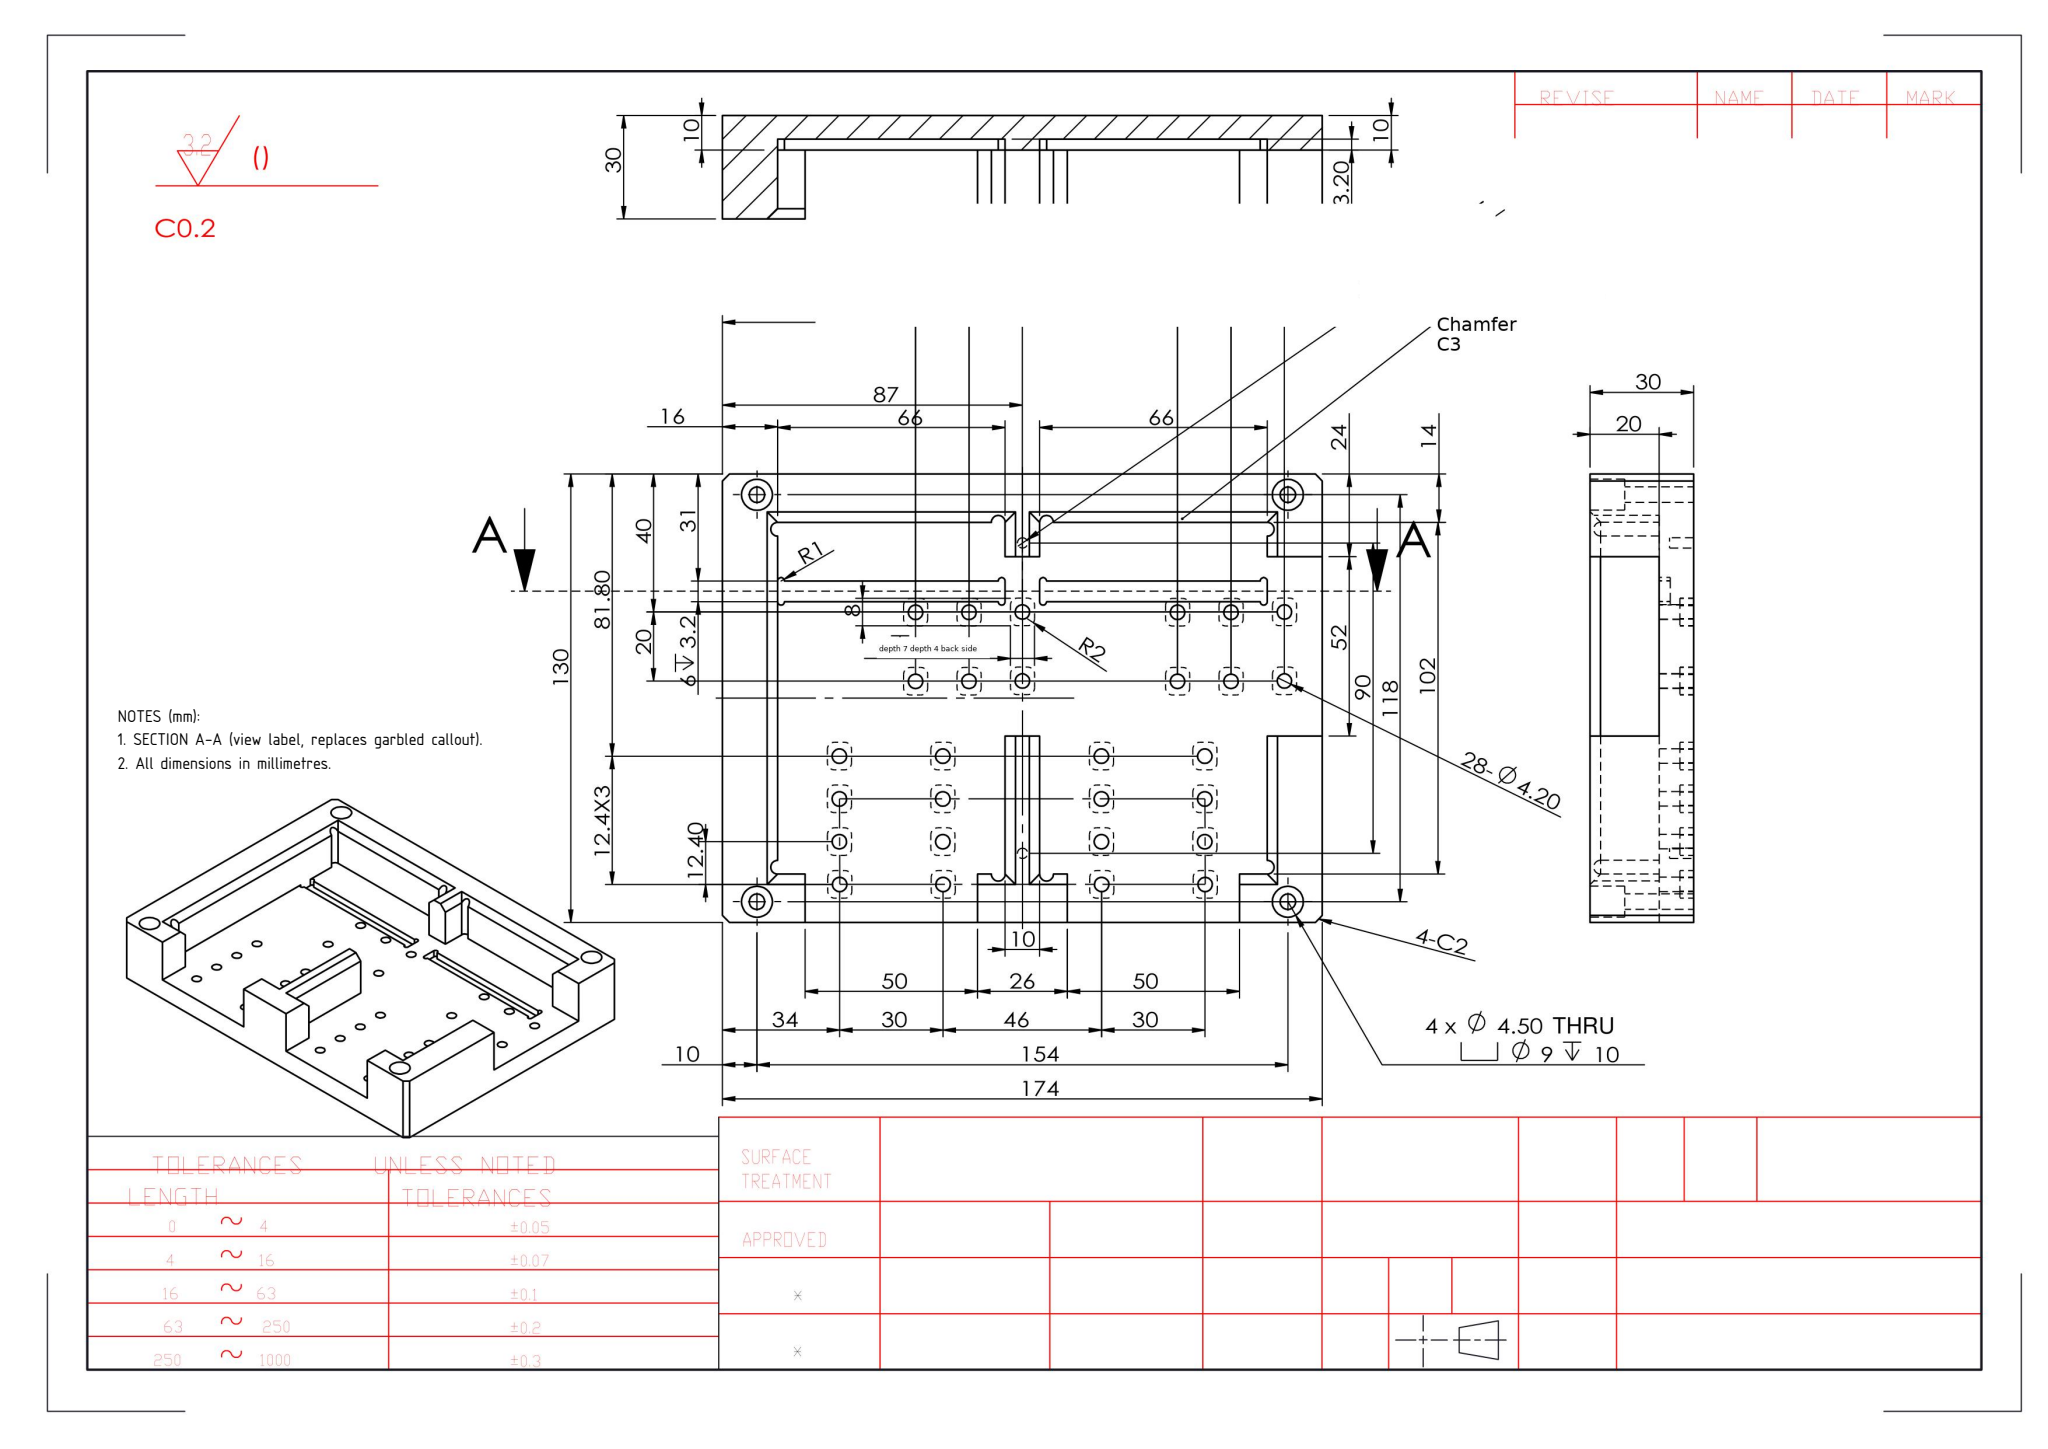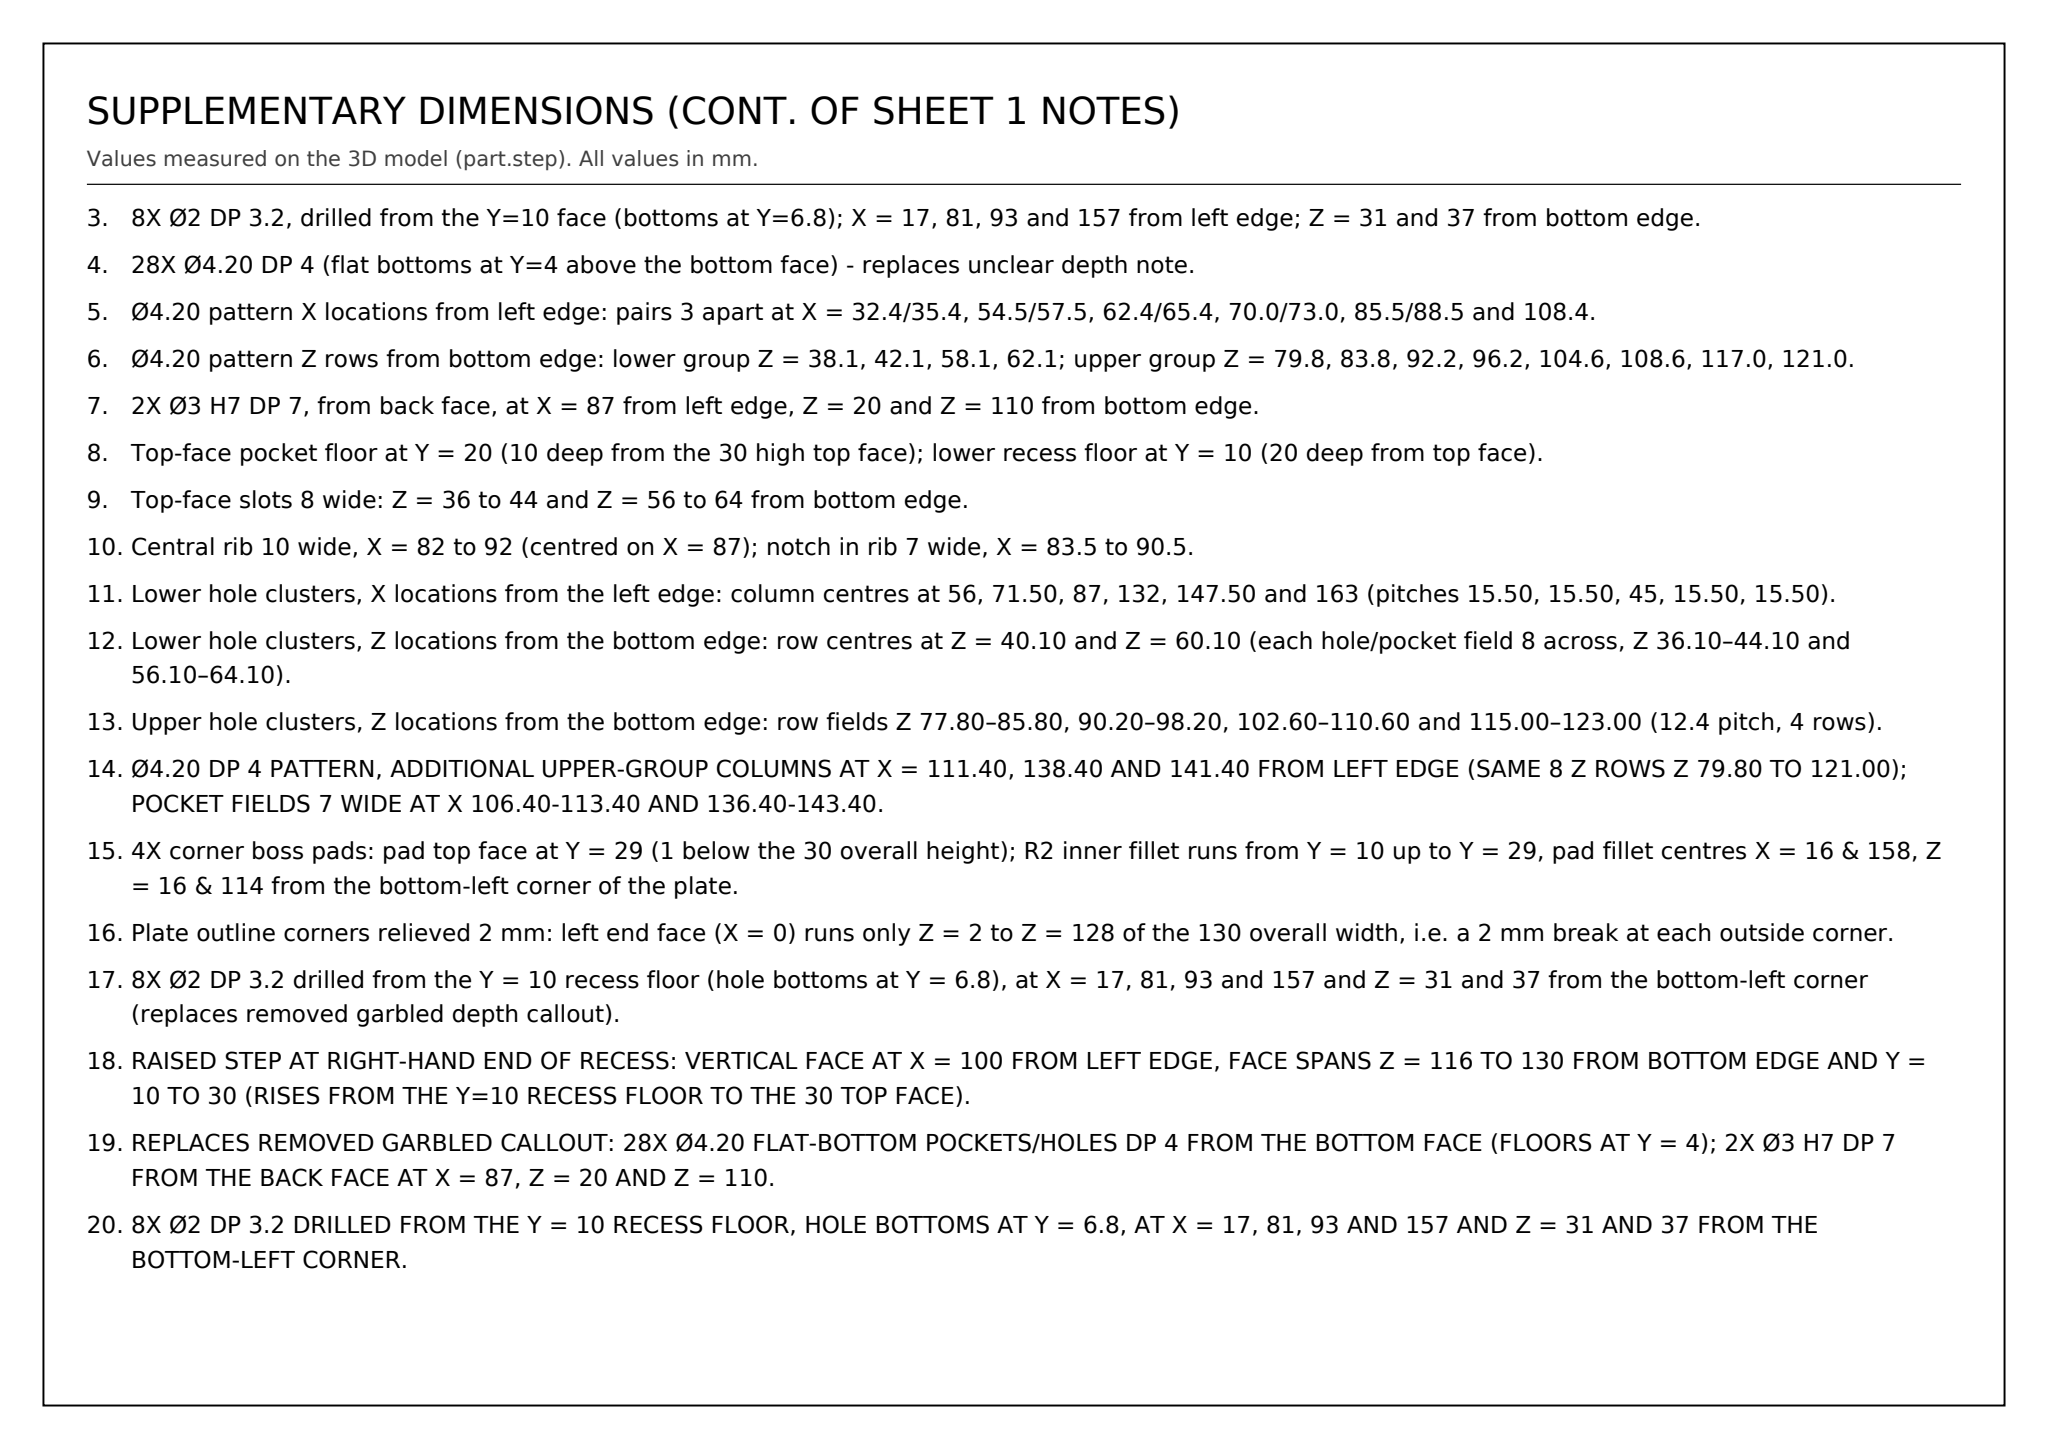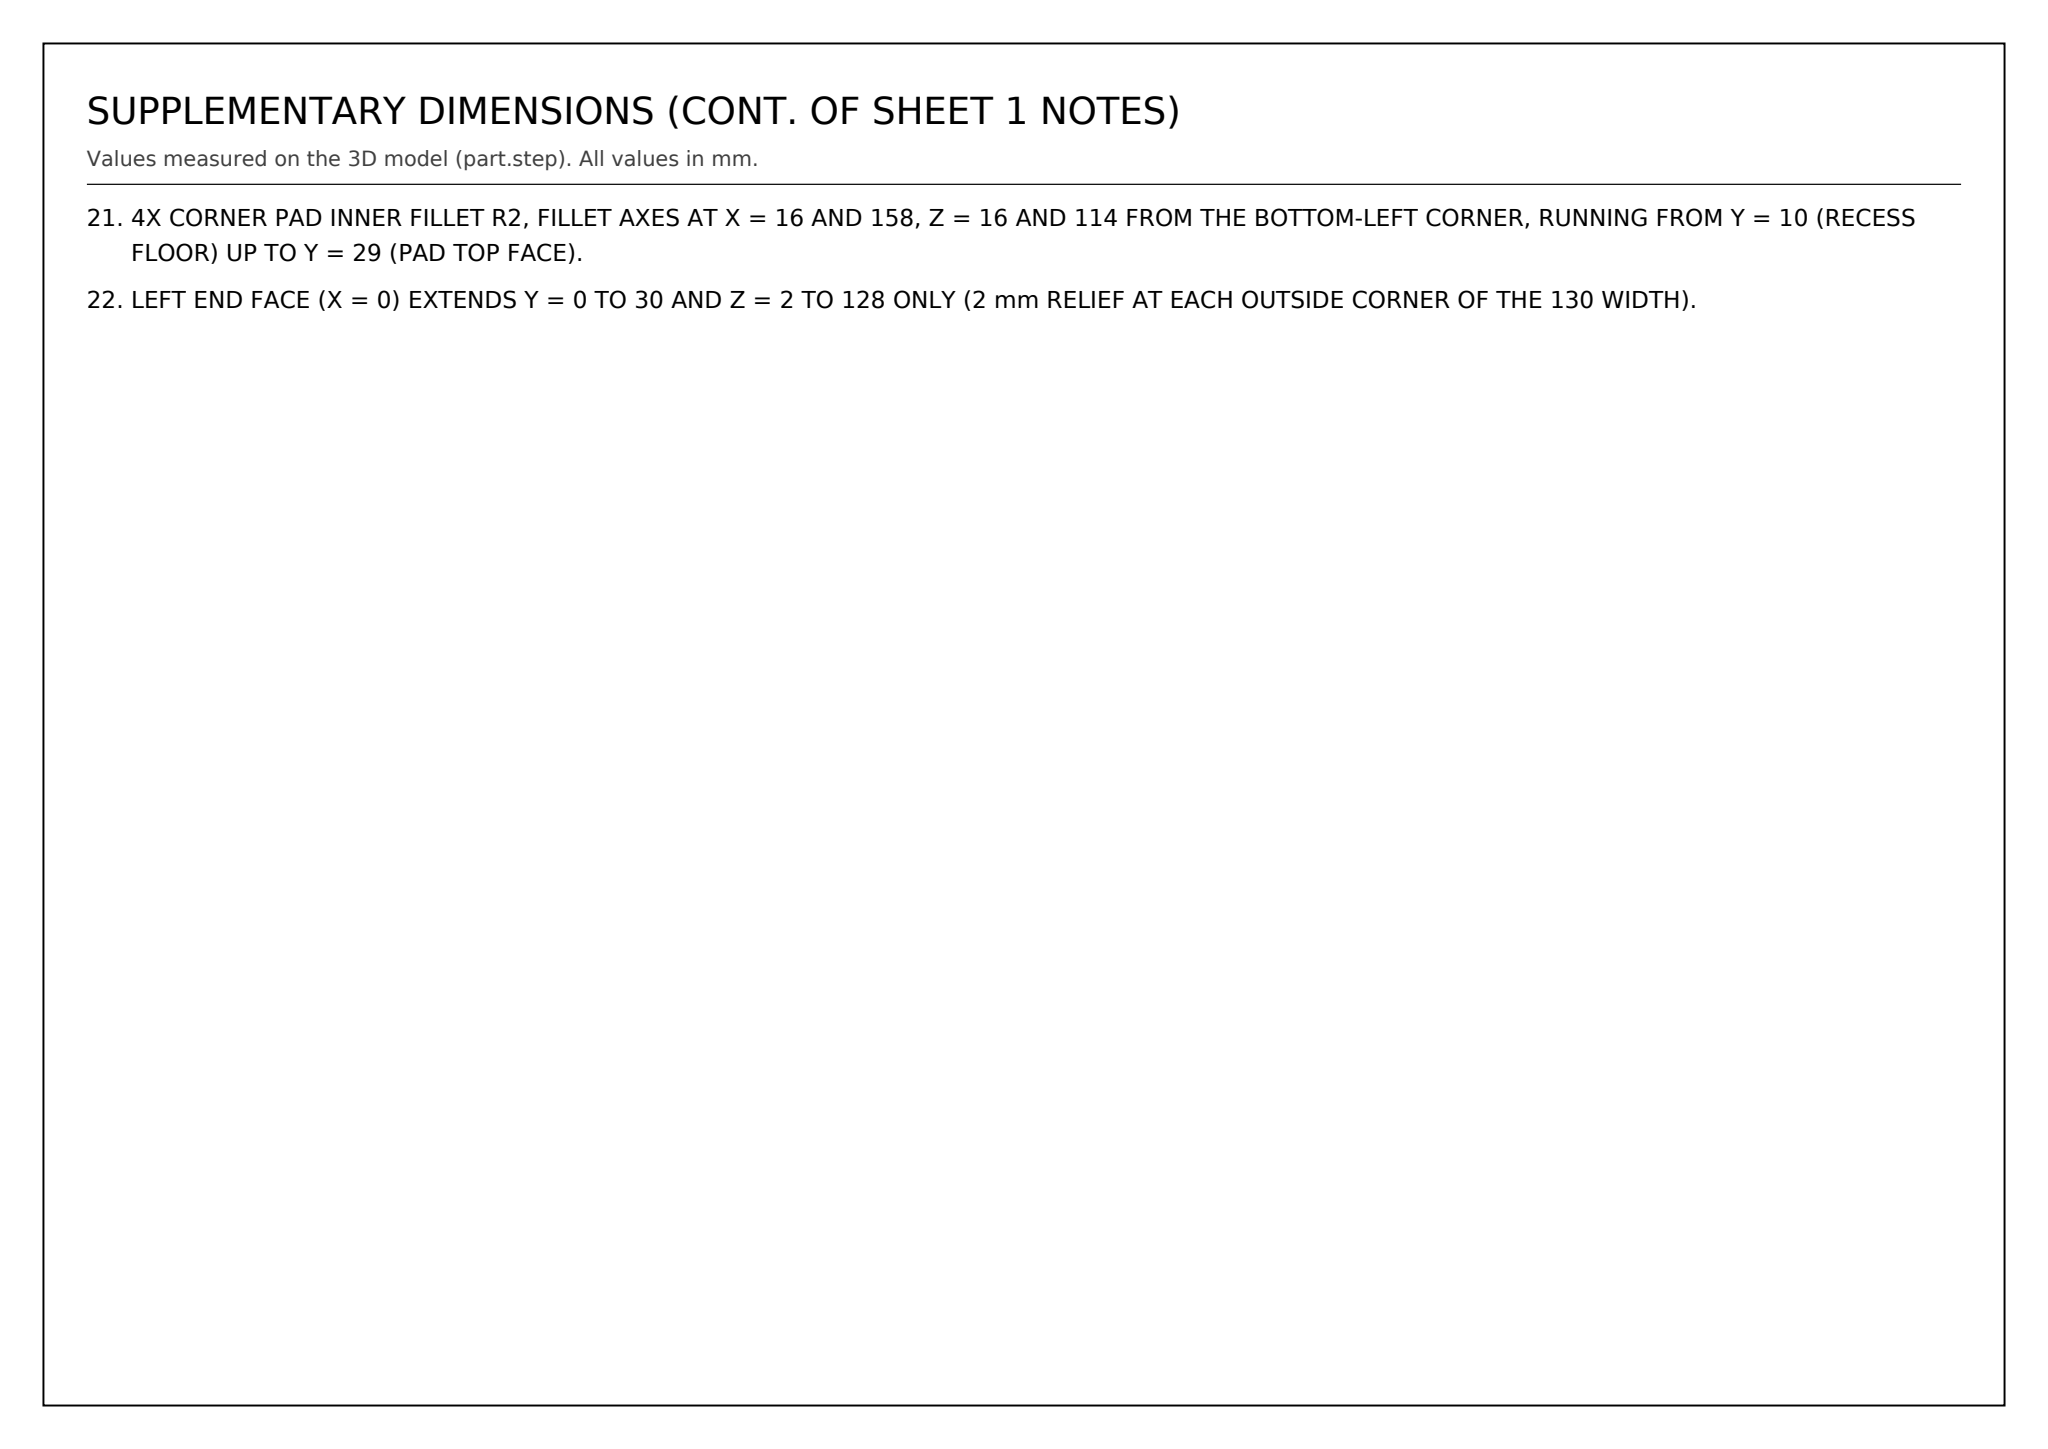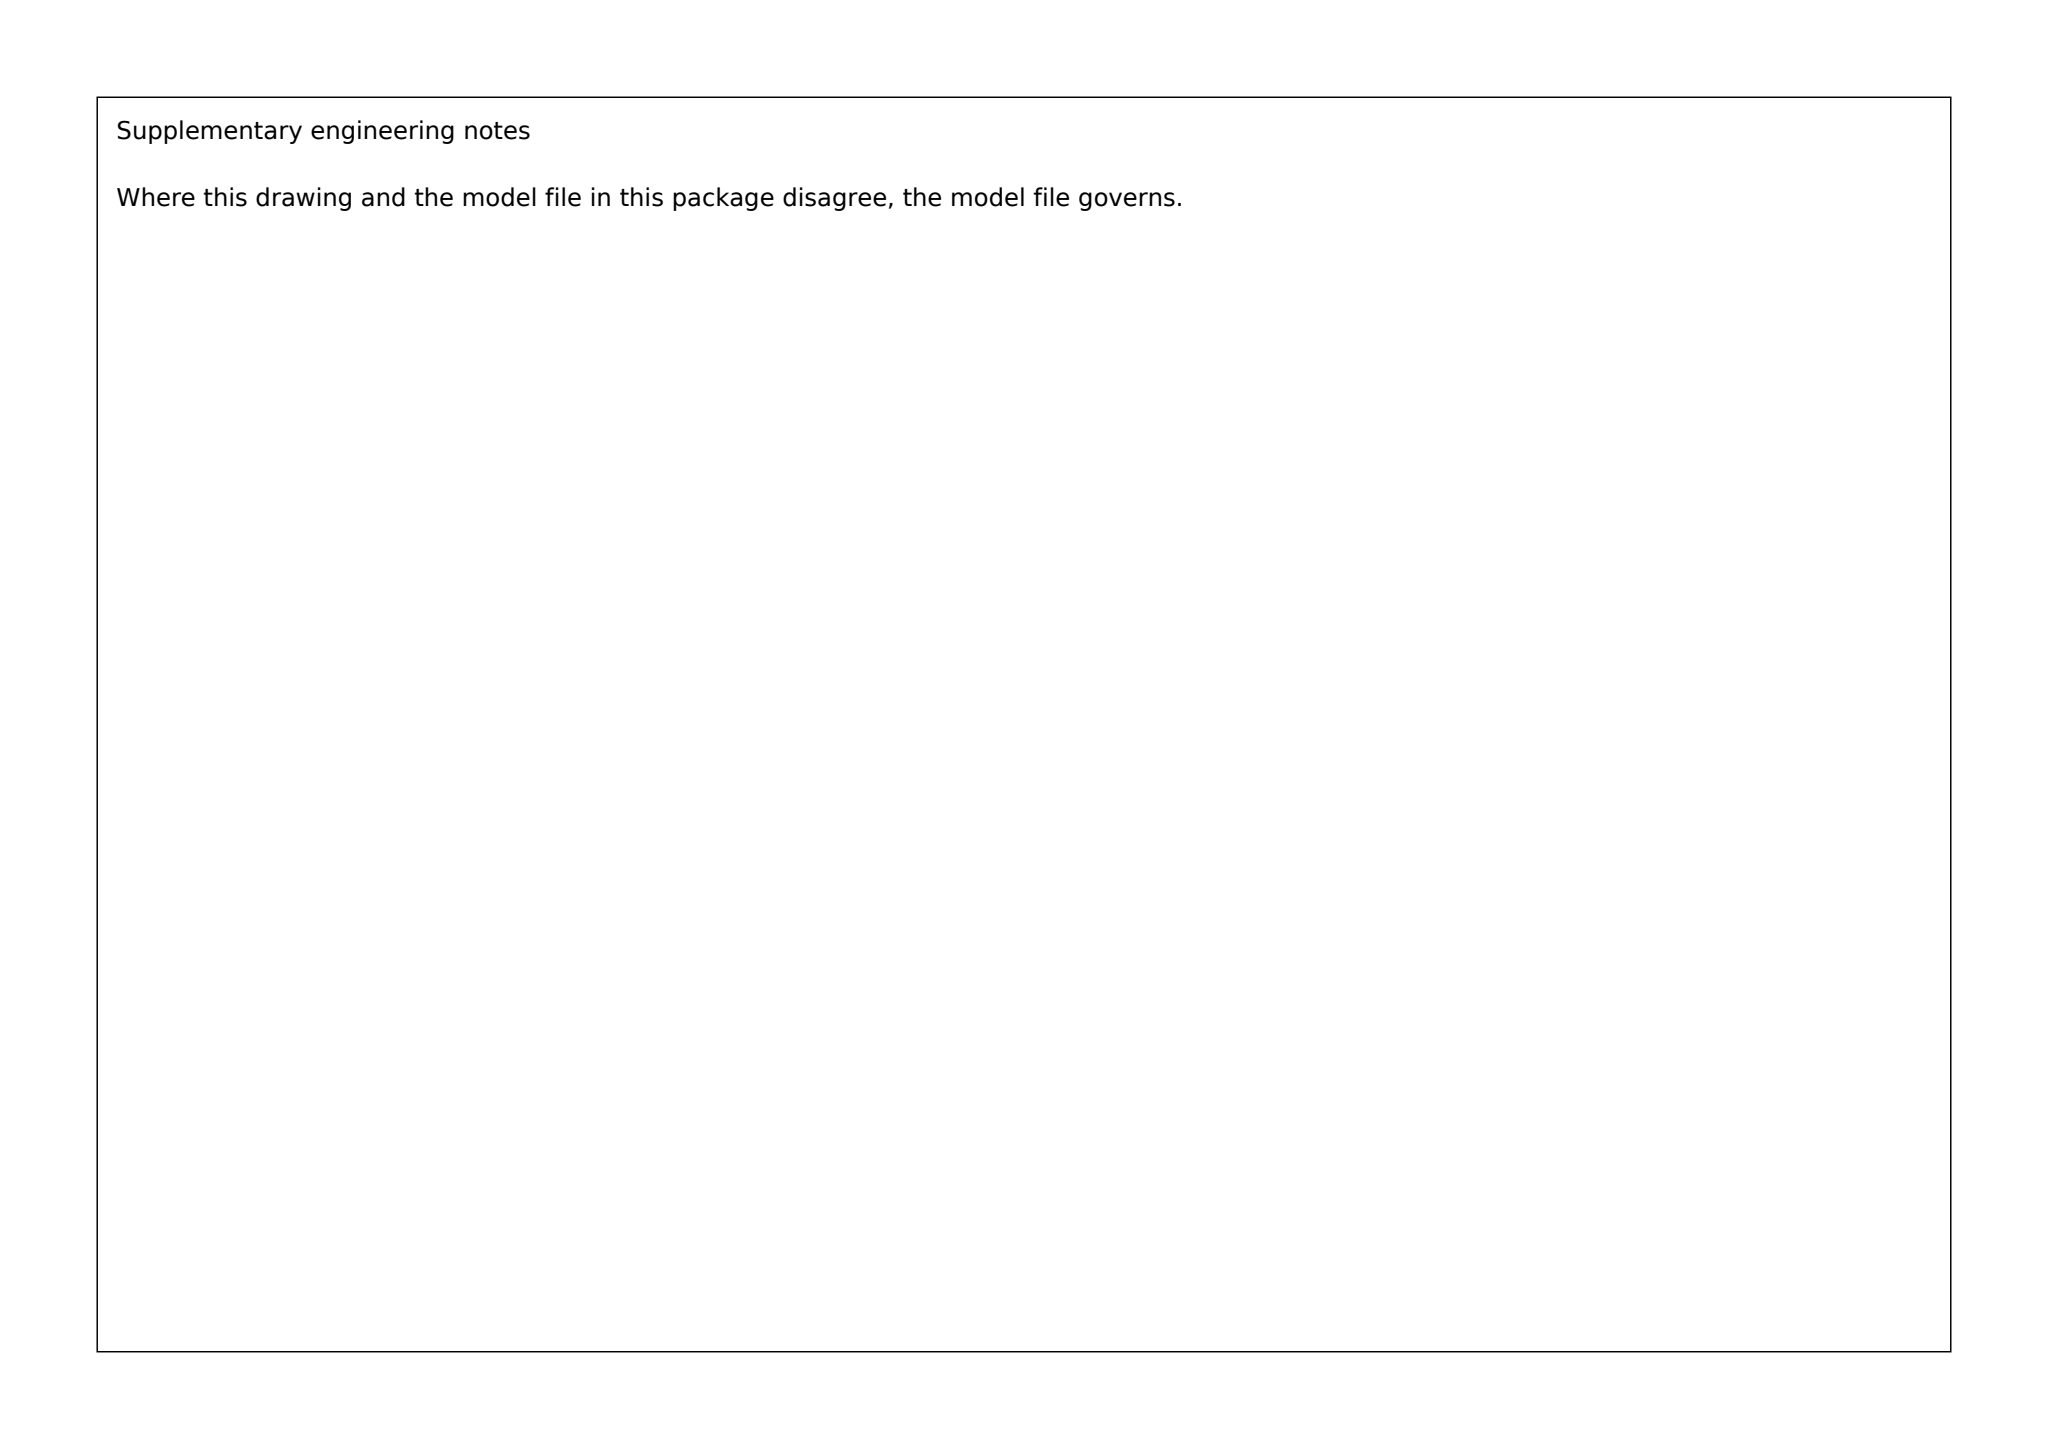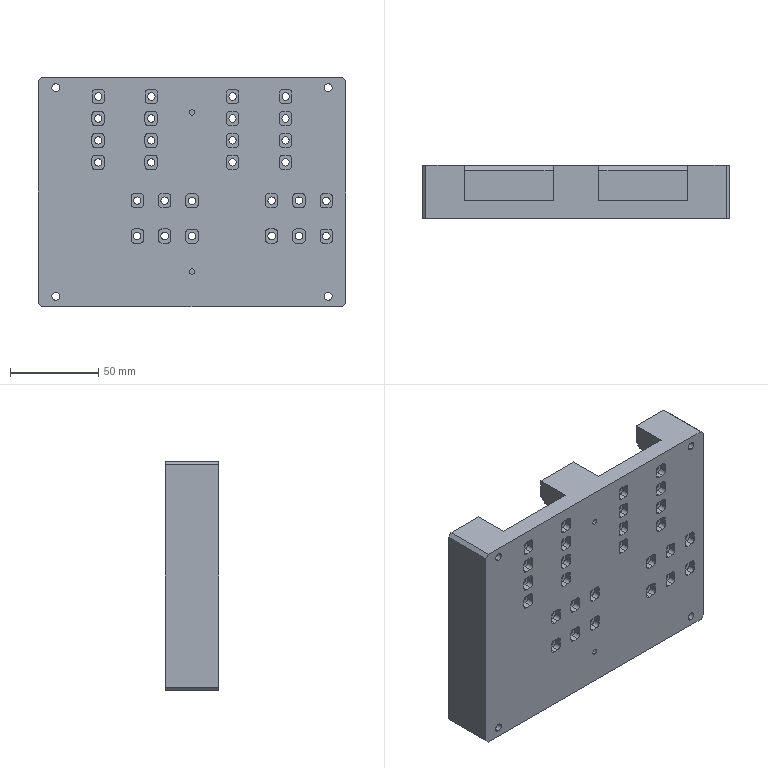Part | SolidWorks | mm | 1 solid | 412 faces | box 174 x 30 x 130 mm | volume 336493 mm3 | cylinder 210 | plane 202 | commonest cylinder face diameters 4 x122 4.2 x56 2 x12 9 x8 4.5 x8 3 x4
Drawing notes:
SECTION A-A (view label, replaces garbled callout). | from the solid: section cut shown in STEP model thickness 30 (bbox_xyz y=30)
All dimensions in millimetres. | from the solid: STEP model facts stated in mm
8X Ø2 DP 3.2, drilled from the Y=10 face (bottoms at Y=6.8); X = 17, 81, 93 and 157 from left edge; Z = 31 and 37 from bottom edge. | from the solid: STEP lists Ø2 y-axis bores (from y=6.8 to y=10) at only 8 locations: (17,31),(17,37),(81,31),(81,37),(93,31),(93,37),(157,31),(157,37) - i.e. 4 X positions x 2 Z positions = 8, not 12.
28X Ø4.20 DP 4 (flat bottoms at Y=4 above the bottom face) - replaces unclear depth note. | from the solid: cylinders dia 4.0 axis y length 4.0; y-plane offset 4.0 count 28
Ø4.20 pattern X locations from left edge: pairs 3 apart at X = 32.4/35.4, 54.5/57.5, 62.4/65.4, 70.0/73.0, 85.5/88.5 and 108.4. | from the solid: cylinders dia 4.0 len 4.0 x-positions 32.4,35.4,54.5,57.5,62.4,65.4,70.0,73.0,85.5,88.5,108.4
Ø4.20 pattern Z rows from bottom edge: lower group Z = 38.1, 42.1, 58.1, 62.1; upper group Z = 79.8, 83.8, 92.2, 96.2, 104.6, 108.6, 117.0, 121.0. | from the solid: cylinders dia 4.0 len 4.0 z-positions 38.1/42.1/58.1/62.1 and 79.8/83.8/92.2/96.2/104.6/108.6/117.0/121.0
2X Ø3 H7 DP 7, from back face, at X = 87 from left edge, Z = 20 and Z = 110 from bottom edge. | from the solid: cylinders dia 3.0 axis y len 7.0 at (87,20) and (87,110); y-plane 7.0 count 2
Top-face pocket floor at Y = 20 (10 deep from the 30 high top face); lower recess floor at Y = 10 (20 deep from top face). | from the solid: y-planes 30.0, 20.0 (count 4), 10.0, 0.0; bbox y = 30
Top-face slots 8 wide: Z = 36 to 44 and Z = 56 to 64 from bottom edge. | from the solid: z-planes 36.0, 37.0, 44.0, 56.0, 64.0 (count 2 each)
Central rib 10 wide, X = 82 to 92 (centred on X = 87); notch in rib 7 wide, X = 83.5 to 90.5. | from the solid: x-planes 82.0 (count 3), 92.0 (count 3), 83.5 (count 2), 90.5 (count 2)
Lower hole clusters, X locations from the left edge: column centres at 56, 71.50, 87, 132, 147.50 and 163 (pitches 15.50, 15.50, 45, 15.50, 15.50). | from the solid: axis_planes x = 52.5/59.5, 68.0/75.0, 83.5/90.5, 128.5/135.5, 144.0/151.0, 159.5/166.5 (7 wide groups, centres 56, 71.5, 87, 132, 147.5, 163)
Lower hole clusters, Z locations from the bottom edge: row centres at Z = 40.10 and Z = 60.10 (each hole/pocket field 8 across, Z 36.10–44.10 and 56.10–64.10). | from the solid: axis_planes z = 36.1, 44.1, 56.1, 64.1 (4 each)
Upper hole clusters, Z locations from the bottom edge: row fields Z 77.80–85.80, 90.20–98.20, 102.60–110.60 and 115.00–123.00 (12.4 pitch, 4 rows). | from the solid: axis_planes z = 77.8, 85.8, 90.2, 98.2, 102.6, 110.6, 115.0, 123.0 (4 each)
Ø4.20 DP 4 PATTERN, ADDITIONAL UPPER-GROUP COLUMNS AT X = 111.40, 138.40 AND 141.40 FROM LEFT EDGE (SAME 8 Z ROWS Z 79.80 TO 121.00); POCKET FIELDS 7 WIDE AT X 106.40-113.40 AND 136.40-143.40. | from the solid: axis_planes x=106.4/113.4 and x=136.4/143.4 pocket-wall pairs, identical 2 mm offsets to the x=30.4/37.4 and x=60.4/67.4 pairs that bracket the listed Ø4.0 (Ø4.20) hole columns x=32.4/35.4 and 62.4/65.4; cylinder dia 4 at x=108.4
4X corner boss pads: pad top face at Y = 29 (1 below the 30 overall height); R2 inner fillet runs from Y = 10 up to Y = 29, pad fillet centres X = 16 & 158, Z = 16 & 114 from the bottom-left corner of the plate. | from the solid: cylinders: concave arc Ø4, axis y, at (16,-,16), (16,-,114), (158,-,16), (158,-,114), from y=10.0 to y=29.0, 180 deg
Plate outline corners relieved 2 mm: left end face (X = 0) runs only Z = 2 to Z = 128 of the 130 overall width, i.e. a 2 mm break at each outside corner. | from the solid: axis_planes: normal x, offset 0.0, extent y 0.0-30.0, z 2.0-128.0
8X Ø2 DP 3.2 drilled from the Y = 10 recess floor (hole bottoms at Y = 6.8), at X = 17, 81, 93 and 157 and Z = 31 and 37 from the bottom-left corner (replaces removed garbled depth callout). | from the solid: cylinders: Ø2, axis y, at (17/81/93/157, -, 31 and 37), from y=6.8 to y=10.0
RAISED STEP AT RIGHT-HAND END OF RECESS: VERTICAL FACE AT X = 100 FROM LEFT EDGE, FACE SPANS Z = 116 TO 130 FROM BOTTOM EDGE AND Y = 10 TO 30 (RISES FROM THE Y=10 RECESS FLOOR TO THE 30 TOP FACE). | from the solid: axis_planes entry: normal x, offset 100.0, extent y [10.0,30.0], z [116.0,130.0], area 275
REPLACES REMOVED GARBLED CALLOUT: 28X Ø4.20 FLAT-BOTTOM POCKETS/HOLES DP 4 FROM THE BOTTOM FACE (FLOORS AT Y = 4); 2X Ø3 H7 DP 7 FROM THE BACK FACE AT X = 87, Z = 20 AND Z = 110. | from the solid: cylinders dia 4.0 axis y, from 0.0 to 4.0 (e.g. at X=108.4/111.4, Z=79.8-121.0); supplementary note 7 for the 2X Ø3 H7 DP 7
8X Ø2 DP 3.2 DRILLED FROM THE Y = 10 RECESS FLOOR, HOLE BOTTOMS AT Y = 6.8, AT X = 17, 81, 93 AND 157 AND Z = 31 AND 37 FROM THE BOTTOM-LEFT CORNER. | from the solid: cylinders dia 2.0 axis y at (17,31),(17,37),(81,31),(81,37),(93,31),(93,37),(157,31),(157,37), from 6.8 to 10.0
4X CORNER PAD INNER FILLET R2, FILLET AXES AT X = 16 AND 158, Z = 16 AND 114 FROM THE BOTTOM-LEFT CORNER, RUNNING FROM Y = 10 (RECESS FLOOR) UP TO Y = 29 (PAD TOP FACE). | from the solid: cylinders dia 4.0 axis y at (16,16),(16,114),(158,16),(158,114), from 10.0 to 29.0, arc 180 deg
LEFT END FACE (X = 0) EXTENDS Y = 0 TO 30 AND Z = 2 TO 128 ONLY (2 mm RELIEF AT EACH OUTSIDE CORNER OF THE 130 WIDTH). | from the solid: axis_planes entry: normal x, offset 0.0, extent y [0.0,30.0], z [2.0,128.0], area 3780
build123d program:
from build123d import *

# Parameters (mm, degrees)
SKETCH1_W                                            = 174
SKETCH1_H                                            = 130
EXTRUDE1_DEPTH                                       = 30
SKETCH2_W                                            = 66
SKETCH2_H                                            = 102
EXTRUDE2_DEPTH                                       = 20
SKETCH3_W                                            = 16.148
SKETCH3_H                                            = 52
SKETCH3_W_2                                          = 16
EXTRUDE3_DEPTH                                       = 20
HOLE_SIZE_ACCORDING_TO_HEXAGON_SOCKET_HE_D           = 4.5
HOLE_SIZE_ACCORDING_TO_HEXAGON_SOCKET_HE_CBORE_D     = 9
HOLE_SIZE_ACCORDING_TO_HEXAGON_SOCKET_HE_CBORE_DEPTH = 10
SKETCH6_R                                            = 1.5
EXTRUDE4_DEPTH                                       = 7
CHAMFER1_SIZE                                        = 2
SKETCH9_R                                            = 2.1
CUT_EXTRUDE2_DEPTH                                   = 144.839
SKETCH10_W                                           = 50
SKETCH10_H                                           = 34.995
SKETCH10_H_2                                         = 28.871
CUT_EXTRUDE3_DEPTH                                   = 20
SKETCH11_R                                           = 2.1
CUT_EXTRUDE4_DEPTH                                   = 144.839
SKETCH12_R                                           = 1.953
CUT_EXTRUDE5_DEPTH                                   = 4
CHAMFER2_SIZE                                        = 3
SKETCH13_R                                           = 2
CUT_EXTRUDE6_DEPTH                                   = 20
SKETCH14_W                                           = 66
SKETCH14_H                                           = 6
CUT_EXTRUDE7_DEPTH                                   = 3.2
SKETCH15_R                                           = 1
CUT_EXTRUDE8_DEPTH                                   = 3.2
SKETCH16_R                                           = 2.1
CUT_EXTRUDE9_DEPTH                                   = 20
CUT_EXTRUDE10_DEPTH                                  = 4
LPATTERN1_COUNT                                      = 2
LPATTERN1_PITCH                                      = 76
SKETCH18_R                                           = 2.1
CUT_EXTRUDE11_DEPTH                                  = 34
CUT_EXTRUDE12_DEPTH                                  = 4
LPATTERN2_COUNT                                      = 2
LPATTERN2_PITCH                                      = 76
LPATTERN3_COUNT                                      = 2
LPATTERN3_PITCH                                      = 12.4
LPATTERN3_COPY_1_SKETCH_R                            = 2.1
LPATTERN3_COPY_1_DEPTH                               = 34
LPATTERN3_COPY_2_DEPTH                               = 4
LPATTERN4_COUNT                                      = 2
LPATTERN4_PITCH                                      = 12.4
LPATTERN4_COPY_1_SKETCH_R                            = 2.1
LPATTERN4_COPY_1_DEPTH                               = 34
LPATTERN4_COPY_2_DEPTH                               = 4
LPATTERN5_COUNT                                      = 2
LPATTERN5_PITCH                                      = 15.5
LPATTERN5_COPY_1_SKETCH_R                            = 2.1
LPATTERN5_COPY_1_DEPTH                               = 20
LPATTERN5_COPY_2_DEPTH                               = 4


with BuildPart() as part:
    # Sketch1 → Extrude1 (new body)
    with BuildSketch(Plane(origin=(0, 0, 0), x_dir=(1, 0, 0), z_dir=(0, 1, 0))):
        with Locations((8.286, 40.879)):
            Rectangle(SKETCH1_W, SKETCH1_H)
    extrude(amount=EXTRUDE1_DEPTH)

    # Sketch2 → Extrude2 (cut)
    with BuildSketch(Plane(origin=(0, 30, 0), x_dir=(-1, 0, 0), z_dir=(0, 1, 0))):
        with Locations((29.714, -40.879)):
            Rectangle(SKETCH2_W, SKETCH2_H)
        with Locations((-46.286, -40.879)):
            Rectangle(SKETCH2_W, SKETCH2_H)
    extrude(amount=-EXTRUDE2_DEPTH, mode=Mode.SUBTRACT)

    # Sketch3 → Extrude3 (cut)
    with BuildSketch(Plane(origin=(0, 30, 0), x_dir=(-1, 0, 0), z_dir=(0, 1, 0))):
        with Locations((-11.36, -55.879)):
            Rectangle(SKETCH3_W, SKETCH3_H)
        with Locations((-87.286, -55.879)):
            Rectangle(SKETCH3_W_2, SKETCH3_H)
    extrude(amount=-EXTRUDE3_DEPTH, mode=Mode.SUBTRACT)

    # Hole Size according to Hexagon Socket He (through all)
    with Locations(Plane(origin=(-68.714, 30, -99.879), x_dir=(0, 0, 1), z_dir=(0, 1, 0))):
        with Locations((0, 0), (0, 154), (118, 154), (118, 0)):
            CounterBoreHole(HOLE_SIZE_ACCORDING_TO_HEXAGON_SOCKET_HE_D / 2, HOLE_SIZE_ACCORDING_TO_HEXAGON_SOCKET_HE_CBORE_D / 2, HOLE_SIZE_ACCORDING_TO_HEXAGON_SOCKET_HE_CBORE_DEPTH)

    # Sketch6 → Extrude4 (cut)
    with BuildSketch(Plane.XZ):
        with Locations(Location((8.286, 4.121, 0), (0, 0, 270))):
            Circle(SKETCH6_R)
        with Locations(Location((8.286, -85.879, 0), (0, 0, 270))):
            Circle(SKETCH6_R)
    extrude(amount=-EXTRUDE4_DEPTH, mode=Mode.SUBTRACT)

    # Chamfer1
    chamfer1_edges = [part.edges().sort_by_distance(p)[0] for p in [
        (-78.714, 15, -105.879),
        (95.286, 15, -105.879),
        (95.286, 15, 24.121),
        (-78.714, 15, 24.121),
    ]]
    chamfer(chamfer1_edges, length=CHAMFER1_SIZE)

    # Sketch9 → Cut-Extrude2 (cut, through all)
    with BuildSketch(Plane(origin=(0, 10, 0), x_dir=(1, 0, 0), z_dir=(0, 1, 0))):
        with Locations(Location((8.286, 65.879, 0), (0, 0, 270))):
            Circle(SKETCH9_R)
        with Locations(Location((8.286, 45.879, 0), (0, 0, 270))):
            Circle(SKETCH9_R)
        with Locations(Location((84.286, 65.879, 0), (0, 0, 270))):
            Circle(SKETCH9_R)
        with Locations(Location((84.286, 45.879, 0), (0, 0, 270))):
            Circle(SKETCH9_R)
    extrude(amount=-CUT_EXTRUDE2_DEPTH, mode=Mode.SUBTRACT)

    # Sketch10 → Cut-Extrude3 (cut)
    with BuildSketch(Plane(origin=(0, 30, 0), x_dir=(1, 0, 0), z_dir=(0, 1, 0))):
        with Locations((-29.714, -18.721)):
            Rectangle(SKETCH10_W, SKETCH10_H)
        with Locations((46.286, -15.659)):
            Rectangle(SKETCH10_W, SKETCH10_H_2)
    extrude(amount=-CUT_EXTRUDE3_DEPTH, mode=Mode.SUBTRACT)

    # Sketch11 → Cut-Extrude4 (cut, through all)
    with BuildSketch(Plane(origin=(0, 10, 0), x_dir=(1, 0, 0), z_dir=(0, 1, 0))):
        with Locations(Location((-44.714, -13.121, 0), (0, 0, 270))):
            Circle(SKETCH11_R)
        with Locations(Location((-14.714, -13.121, 0), (0, 0, 270))):
            Circle(SKETCH11_R)
        with Locations(Location((31.286, -13.121, 0), (0, 0, 270))):
            Circle(SKETCH11_R)
        with Locations(Location((61.286, -13.121, 0), (0, 0, 270))):
            Circle(SKETCH11_R)
    extrude(amount=-CUT_EXTRUDE4_DEPTH, mode=Mode.SUBTRACT)

    # Sketch12 → Cut-Extrude5 (cut)
    # profile 1 of 8: a face of its own
    with BuildSketch(Plane.XZ):
        with BuildLine():
            Line((-46.214, 17.121), (-43.214, 17.121))
            ThreePointArc((-43.214, 17.121), (-41.8, 16.535), (-41.214, 15.121))
            Line((-41.214, 15.121), (-41.214, 11.121))
            ThreePointArc((-41.214, 11.121), (-41.8, 9.706), (-43.214, 9.121))
            Line((-43.214, 9.121), (-46.214, 9.121))
            ThreePointArc((-46.214, 9.121), (-47.629, 9.706), (-48.214, 11.121))
            Line((-48.214, 11.121), (-48.214, 15.121))
            ThreePointArc((-48.214, 15.121), (-47.629, 16.535), (-46.214, 17.121))
        make_face()
        with Locations((-44.714, 13.121)):
            Circle(SKETCH12_R, mode=Mode.SUBTRACT)
    # profile 2 of 8: a face of its own
    with BuildSketch(Plane.XZ):
        with BuildLine():
            Line((6.786, -61.879), (9.786, -61.879))
            ThreePointArc((9.786, -61.879), (11.2, -62.465), (11.786, -63.879))
            Line((11.786, -63.879), (11.786, -67.879))
            ThreePointArc((11.786, -67.879), (11.2, -69.294), (9.786, -69.879))
            Line((9.786, -69.879), (6.786, -69.879))
            ThreePointArc((6.786, -69.879), (5.371, -69.294), (4.786, -67.879))
            Line((4.786, -67.879), (4.786, -63.879))
            ThreePointArc((4.786, -63.879), (5.371, -62.465), (6.786, -61.879))
        make_face()
        with Locations((8.286, -65.879)):
            Circle(SKETCH12_R, mode=Mode.SUBTRACT)
    # profile 3 of 8: a face of its own
    with BuildSketch(Plane.XZ):
        with BuildLine():
            Line((6.786, -41.879), (9.786, -41.879))
            ThreePointArc((9.786, -41.879), (11.2, -42.465), (11.786, -43.879))
            Line((11.786, -43.879), (11.786, -47.879))
            ThreePointArc((11.786, -47.879), (11.2, -49.294), (9.786, -49.879))
            Line((9.786, -49.879), (6.786, -49.879))
            ThreePointArc((6.786, -49.879), (5.371, -49.294), (4.786, -47.879))
            Line((4.786, -47.879), (4.786, -43.879))
            ThreePointArc((4.786, -43.879), (5.371, -42.465), (6.786, -41.879))
        make_face()
        with Locations((8.286, -45.879)):
            Circle(SKETCH12_R, mode=Mode.SUBTRACT)
    # profile 4 of 8: a face of its own
    with BuildSketch(Plane.XZ):
        with BuildLine():
            Line((82.786, -41.879), (85.786, -41.879))
            ThreePointArc((85.786, -41.879), (87.2, -42.465), (87.786, -43.879))
            Line((87.786, -43.879), (87.786, -47.879))
            ThreePointArc((87.786, -47.879), (87.2, -49.294), (85.786, -49.879))
            Line((85.786, -49.879), (82.786, -49.879))
            ThreePointArc((82.786, -49.879), (81.371, -49.294), (80.786, -47.879))
            Line((80.786, -47.879), (80.786, -43.879))
            ThreePointArc((80.786, -43.879), (81.371, -42.465), (82.786, -41.879))
        make_face()
        with Locations((84.286, -45.879)):
            Circle(SKETCH12_R, mode=Mode.SUBTRACT)
    # profile 5 of 8: a face of its own
    with BuildSketch(Plane.XZ):
        with BuildLine():
            Line((82.786, -61.879), (85.786, -61.879))
            ThreePointArc((85.786, -61.879), (87.2, -62.465), (87.786, -63.879))
            Line((87.786, -63.879), (87.786, -67.879))
            ThreePointArc((87.786, -67.879), (87.2, -69.294), (85.786, -69.879))
            Line((85.786, -69.879), (82.786, -69.879))
            ThreePointArc((82.786, -69.879), (81.371, -69.294), (80.786, -67.879))
            Line((80.786, -67.879), (80.786, -63.879))
            ThreePointArc((80.786, -63.879), (81.371, -62.465), (82.786, -61.879))
        make_face()
        with Locations((84.286, -65.879)):
            Circle(SKETCH12_R, mode=Mode.SUBTRACT)
    # profile 6 of 8: a face of its own
    with BuildSketch(Plane.XZ):
        with BuildLine():
            Line((29.786, 17.121), (32.786, 17.121))
            ThreePointArc((32.786, 17.121), (34.2, 16.535), (34.786, 15.121))
            Line((34.786, 15.121), (34.786, 11.121))
            ThreePointArc((34.786, 11.121), (34.2, 9.706), (32.786, 9.121))
            Line((32.786, 9.121), (29.786, 9.121))
            ThreePointArc((29.786, 9.121), (28.371, 9.706), (27.786, 11.121))
            Line((27.786, 11.121), (27.786, 15.121))
            ThreePointArc((27.786, 15.121), (28.371, 16.535), (29.786, 17.121))
        make_face()
        with Locations((31.286, 13.121)):
            Circle(SKETCH12_R, mode=Mode.SUBTRACT)
    # profile 7 of 8: a face of its own
    with BuildSketch(Plane.XZ):
        with BuildLine():
            Line((59.786, 17.121), (62.786, 17.121))
            ThreePointArc((62.786, 17.121), (64.2, 16.535), (64.786, 15.121))
            Line((64.786, 15.121), (64.786, 11.121))
            ThreePointArc((64.786, 11.121), (64.2, 9.706), (62.786, 9.121))
            Line((62.786, 9.121), (59.786, 9.121))
            ThreePointArc((59.786, 9.121), (58.371, 9.706), (57.786, 11.121))
            Line((57.786, 11.121), (57.786, 15.121))
            ThreePointArc((57.786, 15.121), (58.371, 16.535), (59.786, 17.121))
        make_face()
        with Locations((61.286, 13.121)):
            Circle(SKETCH12_R, mode=Mode.SUBTRACT)
    # profile 8 of 8: a face of its own
    with BuildSketch(Plane.XZ):
        with BuildLine():
            Line((-16.214, 17.121), (-13.214, 17.121))
            ThreePointArc((-13.214, 17.121), (-11.8, 16.535), (-11.214, 15.121))
            Line((-11.214, 15.121), (-11.214, 11.121))
            ThreePointArc((-11.214, 11.121), (-11.8, 9.706), (-13.214, 9.121))
            Line((-13.214, 9.121), (-16.214, 9.121))
            ThreePointArc((-16.214, 9.121), (-17.629, 9.706), (-18.214, 11.121))
            Line((-18.214, 11.121), (-18.214, 15.121))
            ThreePointArc((-18.214, 15.121), (-17.629, 16.535), (-16.214, 17.121))
        make_face()
        with Locations((-14.714, 13.121)):
            Circle(SKETCH12_R, mode=Mode.SUBTRACT)
    extrude(amount=-CUT_EXTRUDE5_DEPTH, mode=Mode.SUBTRACT)

    # Chamfer2
    chamfer2_edges = [part.edges().sort_by_distance(p)[0] for p in [
        (-0.7143, 30, 10.121),
        (-62.714, 30, -40.879),
        (-58.714, 30, 10.121),
        (3.286, 30, -9.879),
        (-29.714, 30, -91.879),
        (75.286, 30, 10.121),
        (13.286, 30, -86.879),
        (17.286, 30, 10.121),
        (79.286, 30, -9.879),
        (46.286, 30, -91.879),
        (13.286, 30, -9.879),
        (3.286, 30, -86.879),
        (79.286, 30, -86.879),
    ]]
    chamfer(chamfer2_edges, length=CHAMFER2_SIZE)

    # Sketch13 → Cut-Extrude6 (cut)
    with BuildSketch(Plane(origin=(0, 30, 0), x_dir=(1, 0, 0), z_dir=(0, 1, 0))):
        with Locations((-62.714, 89.879)):
            Circle(SKETCH13_R)
        with Locations((1.286, 91.879)):
            Circle(SKETCH13_R)
        with Locations((-62.714, -8.121)):
            Circle(SKETCH13_R)
        with Locations((1.286, -10.121)):
            Circle(SKETCH13_R)
        with Locations((79.286, -8.121)):
            Circle(SKETCH13_R)
        with Locations((79.286, 89.879)):
            Circle(SKETCH13_R)
        with Locations((15.286, 91.879)):
            Circle(SKETCH13_R)
        with Locations((15.286, -10.121)):
            Circle(SKETCH13_R)
    extrude(amount=-CUT_EXTRUDE6_DEPTH, mode=Mode.SUBTRACT)

    # Sketch14 → Cut-Extrude7 (cut)
    with BuildSketch(Plane(origin=(0, 10, 0), x_dir=(1, 0, 0), z_dir=(0, 1, 0))):
        with Locations((-29.714, 71.879)):
            Rectangle(SKETCH14_W, SKETCH14_H)
        with Locations((46.286, 71.879)):
            Rectangle(SKETCH14_W, SKETCH14_H)
    extrude(amount=-CUT_EXTRUDE7_DEPTH, mode=Mode.SUBTRACT)

    # Sketch15 → Cut-Extrude8 (cut)
    with BuildSketch(Plane(origin=(0, 10, 0), x_dir=(1, 0, 0), z_dir=(0, 1, 0))):
        with Locations((78.286, 74.879)):
            Circle(SKETCH15_R)
        with Locations((78.286, 68.879)):
            Circle(SKETCH15_R)
        with Locations((14.286, 68.879)):
            Circle(SKETCH15_R)
        with Locations((14.286, 74.879)):
            Circle(SKETCH15_R)
        with Locations((2.286, 74.879)):
            Circle(SKETCH15_R)
        with Locations((2.286, 68.879)):
            Circle(SKETCH15_R)
        with Locations((-61.714, 68.879)):
            Circle(SKETCH15_R)
        with Locations((-61.714, 74.879)):
            Circle(SKETCH15_R)
    extrude(amount=-CUT_EXTRUDE8_DEPTH, mode=Mode.SUBTRACT)

    # Sketch16 → Cut-Extrude9 (cut)
    with BuildSketch(Plane(origin=(0, 10, 0), x_dir=(1, 0, 0), z_dir=(0, 1, 0))):
        with Locations(Location((68.786, 65.779, 0), (0, 0, 270))):
            Circle(SKETCH16_R)
        with Locations(Location((68.786, 45.779, 0), (0, 0, 270))):
            Circle(SKETCH16_R)
    cut_extrude9 = extrude(amount=-CUT_EXTRUDE9_DEPTH, mode=Mode.SUBTRACT)

    # Sketch17 → Cut-Extrude10 (cut)
    with BuildSketch(Plane.XZ):
        with BuildLine():
            Line((67.286, -49.779), (70.286, -49.779))
            ThreePointArc((70.286, -49.779), (71.7, -49.194), (72.286, -47.779))
            Line((72.286, -47.779), (72.286, -43.779))
            ThreePointArc((72.286, -43.779), (71.7, -42.365), (70.286, -41.779))
            Line((70.286, -41.779), (67.286, -41.779))
            ThreePointArc((67.286, -41.779), (65.871, -42.365), (65.286, -43.779))
            Line((65.286, -43.779), (65.286, -47.779))
            ThreePointArc((65.286, -47.779), (65.871, -49.194), (67.286, -49.779))
        make_face()
        with BuildLine():
            Line((67.286, -69.779), (70.286, -69.779))
            ThreePointArc((70.286, -69.779), (71.7, -69.194), (72.286, -67.779))
            Line((72.286, -67.779), (72.286, -63.779))
            ThreePointArc((72.286, -63.779), (71.7, -62.365), (70.286, -61.779))
            Line((70.286, -61.779), (67.286, -61.779))
            ThreePointArc((67.286, -61.779), (65.871, -62.365), (65.286, -63.779))
            Line((65.286, -63.779), (65.286, -67.779))
            ThreePointArc((65.286, -67.779), (65.871, -69.194), (67.286, -69.779))
        make_face()
    cut_extrude10 = extrude(amount=-CUT_EXTRUDE10_DEPTH, mode=Mode.SUBTRACT)

    # LPattern1: Cut-Extrude9, Cut-Extrude10 ×2
    with Locations(*[(-i * LPATTERN1_PITCH, 0, 0) for i in range(1, LPATTERN1_COUNT)]):
        add(cut_extrude9, mode=Mode.SUBTRACT)
        add(cut_extrude10, mode=Mode.SUBTRACT)

    # Sketch18 → Cut-Extrude11 (cut)
    with BuildSketch(Plane(origin=(0, 10, 0), x_dir=(1, 0, 0), z_dir=(0, 1, 0))):
        with Locations(Location((31.186, 11.679, 0), (0, 0, 270))):
            Circle(SKETCH18_R)
        with Locations(Location((61.186, 11.679, 0), (0, 0, 270))):
            Circle(SKETCH18_R)
    cut_extrude11 = extrude(amount=-CUT_EXTRUDE11_DEPTH, mode=Mode.SUBTRACT)

    # Sketch19 → Cut-Extrude12 (cut)
    with BuildSketch(Plane.XZ):
        with BuildLine():
            Line((59.686, -7.679), (62.686, -7.679))
            ThreePointArc((62.686, -7.679), (64.1, -8.265), (64.686, -9.679))
            Line((64.686, -9.679), (64.686, -13.679))
            ThreePointArc((64.686, -13.679), (64.1, -15.094), (62.686, -15.679))
            Line((62.686, -15.679), (59.686, -15.679))
            ThreePointArc((59.686, -15.679), (58.271, -15.094), (57.686, -13.679))
            Line((57.686, -13.679), (57.686, -9.679))
            ThreePointArc((57.686, -9.679), (58.271, -8.265), (59.686, -7.679))
        make_face()
        with BuildLine():
            Line((29.686, -15.679), (32.686, -15.679))
            ThreePointArc((32.686, -15.679), (34.1, -15.094), (34.686, -13.679))
            Line((34.686, -13.679), (34.686, -9.679))
            ThreePointArc((34.686, -9.679), (34.1, -8.265), (32.686, -7.679))
            Line((32.686, -7.679), (29.686, -7.679))
            ThreePointArc((29.686, -7.679), (28.271, -8.265), (27.686, -9.679))
            Line((27.686, -9.679), (27.686, -13.679))
            ThreePointArc((27.686, -13.679), (28.271, -15.094), (29.686, -15.679))
        make_face()
    cut_extrude12 = extrude(amount=-CUT_EXTRUDE12_DEPTH, mode=Mode.SUBTRACT)

    # LPattern2: Cut-Extrude11, Cut-Extrude12 ×2
    with Locations(*[(-i * LPATTERN2_PITCH, 0, 0) for i in range(1, LPATTERN2_COUNT)]):
        add(cut_extrude11, mode=Mode.SUBTRACT)
        add(cut_extrude12, mode=Mode.SUBTRACT)

    # LPattern3: Cut-Extrude11, Cut-Extrude12 ×2
    with Locations(*[(0, 0, i * LPATTERN3_PITCH) for i in range(1, LPATTERN3_COUNT)]):
        add(cut_extrude11, mode=Mode.SUBTRACT)
        add(cut_extrude12, mode=Mode.SUBTRACT)

    # LPattern3 copy 1 sketch → LPattern3 copy 1 (cut)
    with BuildSketch(Plane(origin=(-76, 10, 12.4), x_dir=(1, 0, 0), z_dir=(0, 1, 0))):
        with Locations(Location((31.186, 11.679, 0), (0, 0, 270))):
            Circle(LPATTERN3_COPY_1_SKETCH_R)
        with Locations(Location((61.186, 11.679, 0), (0, 0, 270))):
            Circle(LPATTERN3_COPY_1_SKETCH_R)
    extrude(amount=-LPATTERN3_COPY_1_DEPTH, mode=Mode.SUBTRACT)

    # LPattern3 copy 2 sketch → LPattern3 copy 2 (cut)
    with BuildSketch(Plane(origin=(-76, 0, 12.4), x_dir=(1, 0, 0), z_dir=(0, -1, 0))):
        with BuildLine():
            Line((59.686, -7.679), (62.686, -7.679))
            ThreePointArc((62.686, -7.679), (64.1, -8.265), (64.686, -9.679))
            Line((64.686, -9.679), (64.686, -13.679))
            ThreePointArc((64.686, -13.679), (64.1, -15.094), (62.686, -15.679))
            Line((62.686, -15.679), (59.686, -15.679))
            ThreePointArc((59.686, -15.679), (58.271, -15.094), (57.686, -13.679))
            Line((57.686, -13.679), (57.686, -9.679))
            ThreePointArc((57.686, -9.679), (58.271, -8.265), (59.686, -7.679))
        make_face()
        with BuildLine():
            Line((29.686, -15.679), (32.686, -15.679))
            ThreePointArc((32.686, -15.679), (34.1, -15.094), (34.686, -13.679))
            Line((34.686, -13.679), (34.686, -9.679))
            ThreePointArc((34.686, -9.679), (34.1, -8.265), (32.686, -7.679))
            Line((32.686, -7.679), (29.686, -7.679))
            ThreePointArc((29.686, -7.679), (28.271, -8.265), (27.686, -9.679))
            Line((27.686, -9.679), (27.686, -13.679))
            ThreePointArc((27.686, -13.679), (28.271, -15.094), (29.686, -15.679))
        make_face()
    extrude(amount=-LPATTERN3_COPY_2_DEPTH, mode=Mode.SUBTRACT)

    # LPattern4: Cut-Extrude11, Cut-Extrude12 ×2
    with Locations(*[(0, 0, -i * LPATTERN4_PITCH) for i in range(1, LPATTERN4_COUNT)]):
        add(cut_extrude11, mode=Mode.SUBTRACT)
        add(cut_extrude12, mode=Mode.SUBTRACT)

    # LPattern4 copy 1 sketch → LPattern4 copy 1 (cut)
    with BuildSketch(Plane(origin=(-76, 10, -12.4), x_dir=(1, 0, 0), z_dir=(0, 1, 0))):
        with Locations(Location((31.186, 11.679, 0), (0, 0, 270))):
            Circle(LPATTERN4_COPY_1_SKETCH_R)
        with Locations(Location((61.186, 11.679, 0), (0, 0, 270))):
            Circle(LPATTERN4_COPY_1_SKETCH_R)
    extrude(amount=-LPATTERN4_COPY_1_DEPTH, mode=Mode.SUBTRACT)

    # LPattern4 copy 2 sketch → LPattern4 copy 2 (cut)
    with BuildSketch(Plane(origin=(-76, 0, -12.4), x_dir=(1, 0, 0), z_dir=(0, -1, 0))):
        with BuildLine():
            Line((59.686, -7.679), (62.686, -7.679))
            ThreePointArc((62.686, -7.679), (64.1, -8.265), (64.686, -9.679))
            Line((64.686, -9.679), (64.686, -13.679))
            ThreePointArc((64.686, -13.679), (64.1, -15.094), (62.686, -15.679))
            Line((62.686, -15.679), (59.686, -15.679))
            ThreePointArc((59.686, -15.679), (58.271, -15.094), (57.686, -13.679))
            Line((57.686, -13.679), (57.686, -9.679))
            ThreePointArc((57.686, -9.679), (58.271, -8.265), (59.686, -7.679))
        make_face()
        with BuildLine():
            Line((29.686, -15.679), (32.686, -15.679))
            ThreePointArc((32.686, -15.679), (34.1, -15.094), (34.686, -13.679))
            Line((34.686, -13.679), (34.686, -9.679))
            ThreePointArc((34.686, -9.679), (34.1, -8.265), (32.686, -7.679))
            Line((32.686, -7.679), (29.686, -7.679))
            ThreePointArc((29.686, -7.679), (28.271, -8.265), (27.686, -9.679))
            Line((27.686, -9.679), (27.686, -13.679))
            ThreePointArc((27.686, -13.679), (28.271, -15.094), (29.686, -15.679))
        make_face()
    extrude(amount=-LPATTERN4_COPY_2_DEPTH, mode=Mode.SUBTRACT)

    # LPattern5: Cut-Extrude9, Cut-Extrude10 ×2
    with Locations(*[(-i * LPATTERN5_PITCH, 0, 0) for i in range(1, LPATTERN5_COUNT)]):
        add(cut_extrude9, mode=Mode.SUBTRACT)
        add(cut_extrude10, mode=Mode.SUBTRACT)

    # LPattern5 copy 1 sketch → LPattern5 copy 1 (cut)
    with BuildSketch(Plane(origin=(-91.5, 10, 0), x_dir=(1, 0, 0), z_dir=(0, 1, 0))):
        with Locations(Location((68.786, 65.779, 0), (0, 0, 270))):
            Circle(LPATTERN5_COPY_1_SKETCH_R)
        with Locations(Location((68.786, 45.779, 0), (0, 0, 270))):
            Circle(LPATTERN5_COPY_1_SKETCH_R)
    extrude(amount=-LPATTERN5_COPY_1_DEPTH, mode=Mode.SUBTRACT)

    # LPattern5 copy 2 sketch → LPattern5 copy 2 (cut)
    with BuildSketch(Plane(origin=(-91.5, 0, 0), x_dir=(1, 0, 0), z_dir=(0, -1, 0))):
        with BuildLine():
            Line((67.286, -49.779), (70.286, -49.779))
            ThreePointArc((70.286, -49.779), (71.7, -49.194), (72.286, -47.779))
            Line((72.286, -47.779), (72.286, -43.779))
            ThreePointArc((72.286, -43.779), (71.7, -42.365), (70.286, -41.779))
            Line((70.286, -41.779), (67.286, -41.779))
            ThreePointArc((67.286, -41.779), (65.871, -42.365), (65.286, -43.779))
            Line((65.286, -43.779), (65.286, -47.779))
            ThreePointArc((65.286, -47.779), (65.871, -49.194), (67.286, -49.779))
        make_face()
        with BuildLine():
            Line((67.286, -69.779), (70.286, -69.779))
            ThreePointArc((70.286, -69.779), (71.7, -69.194), (72.286, -67.779))
            Line((72.286, -67.779), (72.286, -63.779))
            ThreePointArc((72.286, -63.779), (71.7, -62.365), (70.286, -61.779))
            Line((70.286, -61.779), (67.286, -61.779))
            ThreePointArc((67.286, -61.779), (65.871, -62.365), (65.286, -63.779))
            Line((65.286, -63.779), (65.286, -67.779))
            ThreePointArc((65.286, -67.779), (65.871, -69.194), (67.286, -69.779))
        make_face()
    extrude(amount=-LPATTERN5_COPY_2_DEPTH, mode=Mode.SUBTRACT)


solid = part.part